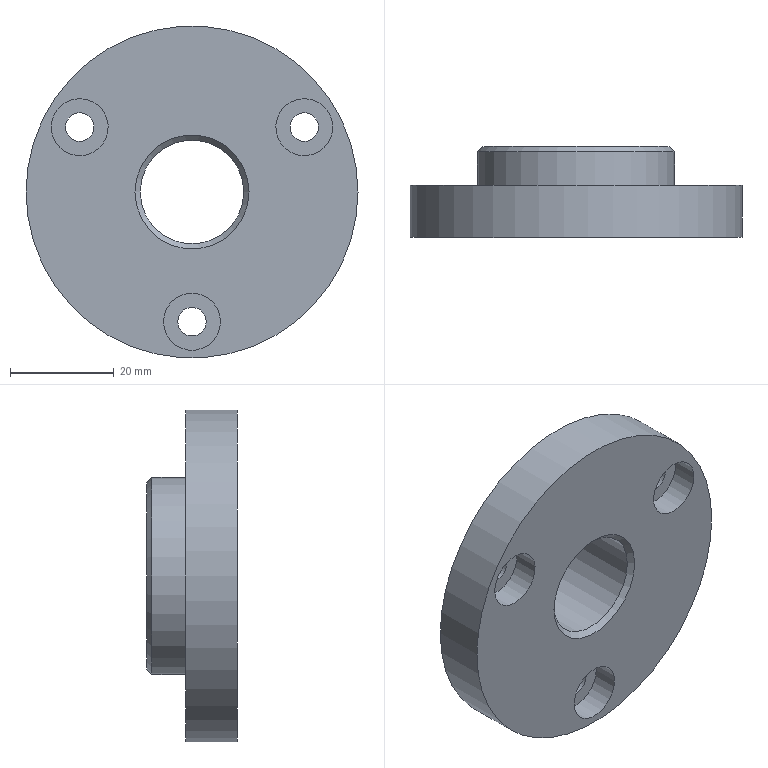Component | NX | FLANGE_COVER | 1 solid | 18 faces | box 64 x 17.5 x 64 mm | volume 33273 mm3 | cylinder 9 | plane 6 | cone 3 | commonest cylinder face diameters 11 x3 5.5 x3 64 x1 38 x1 20 x1
STEP:
#1=CARTESIAN_POINT('',(0.,0.,0.));
#2=DIRECTION('',(0.,0.,1.));
#3=DIRECTION('',(1.,0.,0.));
#4=AXIS2_PLACEMENT_3D('',#1,#2,#3);
#5=CARTESIAN_POINT('',(-127.326,-180.11,50.));
#6=VERTEX_POINT('',#5);
#7=CARTESIAN_POINT('',(-95.326,-180.11,50.));
#8=DIRECTION('',(0.,1.,0.));
#9=DIRECTION('',(-1.,0.,0.));
#10=AXIS2_PLACEMENT_3D('',#7,#8,#9);
#11=CIRCLE('',#10,32.);
#12=CARTESIAN_POINT('',(-95.326,-180.11,50.));
#13=DIRECTION('',(0.,-1.,0.));
#14=DIRECTION('',(1.,0.,0.));
#15=AXIS2_PLACEMENT_3D('',#12,#13,#14);
#16=CYLINDRICAL_SURFACE('',#15,32.);
#17=CARTESIAN_POINT('',(9.425,0.));
#18=DIRECTION('',(-1.,0.));
#19=VECTOR('',#18,1.);
#20=LINE('',#17,#19);
#21=(GEOMETRIC_REPRESENTATION_CONTEXT(2)PARAMETRIC_REPRESENTATION_CONTEXT()REPRESENTATION_CONTEXT('',''));
#22=DEFINITIONAL_REPRESENTATION('',(#20),#21);
#23=PCURVE('',#16,#22);
#24=CARTESIAN_POINT('',(-95.326,-180.11,50.));
#25=DIRECTION('',(0.,1.,0.));
#26=DIRECTION('',(-1.,0.,0.));
#27=AXIS2_PLACEMENT_3D('',#24,#25,#26);
#28=PLANE('',#27);
#29=CARTESIAN_POINT('',(0.,0.));
#30=DIRECTION('',(1.,0.));
#31=AXIS2_PLACEMENT_2D('',#29,#30);
#32=CIRCLE('',#31,32.);
#33=(GEOMETRIC_REPRESENTATION_CONTEXT(2)PARAMETRIC_REPRESENTATION_CONTEXT()REPRESENTATION_CONTEXT('',''));
#34=DEFINITIONAL_REPRESENTATION('',(#32),#33);
#35=PCURVE('',#28,#34);
#36=SURFACE_CURVE('',#11,(#23,#35),.PCURVE_S1.);
#37=EDGE_CURVE('',#6,#6,#36,.T.);
#38=ORIENTED_EDGE('',*,*,#37,.F.);
#39=CARTESIAN_POINT('',(-127.326,-190.11,50.));
#40=VERTEX_POINT('',#39);
#41=CARTESIAN_POINT('',(-127.326,-180.11,50.));
#42=CARTESIAN_POINT('',(-127.326,-190.11,50.));
#43=B_SPLINE_CURVE_WITH_KNOTS('',1,(#41,#42),.UNSPECIFIED.,.F.,.F.,(2,2),(0.,10.),.PIECEWISE_BEZIER_KNOTS.);
#44=CARTESIAN_POINT('',(9.425,0.));
#45=DIRECTION('',(0.,1.));
#46=VECTOR('',#45,1.);
#47=LINE('',#44,#46);
#48=(GEOMETRIC_REPRESENTATION_CONTEXT(2)PARAMETRIC_REPRESENTATION_CONTEXT()REPRESENTATION_CONTEXT('',''));
#49=DEFINITIONAL_REPRESENTATION('',(#47),#48);
#50=PCURVE('',#16,#49);
#51=CARTESIAN_POINT('',(3.142,0.));
#52=DIRECTION('',(0.,1.));
#53=VECTOR('',#52,1.);
#54=LINE('',#51,#53);
#55=(GEOMETRIC_REPRESENTATION_CONTEXT(2)PARAMETRIC_REPRESENTATION_CONTEXT()REPRESENTATION_CONTEXT('',''));
#56=DEFINITIONAL_REPRESENTATION('',(#54),#55);
#57=PCURVE('',#16,#56);
#58=SEAM_CURVE('',#43,(#50,#57),.PCURVE_S1.);
#59=EDGE_CURVE('',#6,#40,#58,.T.);
#60=ORIENTED_EDGE('',*,*,#59,.T.);
#61=CARTESIAN_POINT('',(-95.326,-190.11,50.));
#62=DIRECTION('',(0.,1.,0.));
#63=DIRECTION('',(-1.,0.,0.));
#64=AXIS2_PLACEMENT_3D('',#61,#62,#63);
#65=CIRCLE('',#64,32.);
#66=CARTESIAN_POINT('',(9.425,10.));
#67=DIRECTION('',(-1.,0.));
#68=VECTOR('',#67,1.);
#69=LINE('',#66,#68);
#70=(GEOMETRIC_REPRESENTATION_CONTEXT(2)PARAMETRIC_REPRESENTATION_CONTEXT()REPRESENTATION_CONTEXT('',''));
#71=DEFINITIONAL_REPRESENTATION('',(#69),#70);
#72=PCURVE('',#16,#71);
#73=CARTESIAN_POINT('',(-95.326,-190.11,50.));
#74=DIRECTION('',(0.,1.,0.));
#75=DIRECTION('',(-1.,0.,0.));
#76=AXIS2_PLACEMENT_3D('',#73,#74,#75);
#77=PLANE('',#76);
#78=CARTESIAN_POINT('',(0.,0.));
#79=DIRECTION('',(1.,0.));
#80=AXIS2_PLACEMENT_2D('',#78,#79);
#81=CIRCLE('',#80,32.);
#82=(GEOMETRIC_REPRESENTATION_CONTEXT(2)PARAMETRIC_REPRESENTATION_CONTEXT()REPRESENTATION_CONTEXT('',''));
#83=DEFINITIONAL_REPRESENTATION('',(#81),#82);
#84=PCURVE('',#77,#83);
#85=SURFACE_CURVE('',#65,(#72,#84),.PCURVE_S1.);
#86=EDGE_CURVE('',#40,#40,#85,.T.);
#87=ORIENTED_EDGE('',*,*,#86,.T.);
#88=ORIENTED_EDGE('',*,*,#59,.F.);
#89=EDGE_LOOP('',(#38,#60,#87,#88));
#90=FACE_BOUND('',#89,.T.);
#91=ADVANCED_FACE('',(#90),#16,.T.);
#92=CARTESIAN_POINT('',(-98.076,-180.11,25.));
#93=VERTEX_POINT('',#92);
#94=CARTESIAN_POINT('',(-95.326,-180.11,25.));
#95=DIRECTION('',(0.,1.,0.));
#96=DIRECTION('',(-1.,0.,0.));
#97=AXIS2_PLACEMENT_3D('',#94,#95,#96);
#98=CIRCLE('',#97,2.75);
#99=CARTESIAN_POINT('',(0.,-25.));
#100=DIRECTION('',(1.,0.));
#101=AXIS2_PLACEMENT_2D('',#99,#100);
#102=CIRCLE('',#101,2.75);
#103=(GEOMETRIC_REPRESENTATION_CONTEXT(2)PARAMETRIC_REPRESENTATION_CONTEXT()REPRESENTATION_CONTEXT('',''));
#104=DEFINITIONAL_REPRESENTATION('',(#102),#103);
#105=PCURVE('',#28,#104);
#106=CARTESIAN_POINT('',(-95.326,-148.11,25.));
#107=DIRECTION('',(0.,-1.,0.));
#108=DIRECTION('',(1.,0.,0.));
#109=AXIS2_PLACEMENT_3D('',#106,#107,#108);
#110=CYLINDRICAL_SURFACE('',#109,2.75);
#111=CARTESIAN_POINT('',(9.425,32.));
#112=DIRECTION('',(-1.,0.));
#113=VECTOR('',#112,1.);
#114=LINE('',#111,#113);
#115=(GEOMETRIC_REPRESENTATION_CONTEXT(2)PARAMETRIC_REPRESENTATION_CONTEXT()REPRESENTATION_CONTEXT('',''));
#116=DEFINITIONAL_REPRESENTATION('',(#114),#115);
#117=PCURVE('',#110,#116);
#118=SURFACE_CURVE('',#98,(#105,#117),.PCURVE_S1.);
#119=EDGE_CURVE('',#93,#93,#118,.T.);
#120=ORIENTED_EDGE('',*,*,#119,.F.);
#121=EDGE_LOOP('',(#120));
#122=FACE_BOUND('',#121,.T.);
#123=CARTESIAN_POINT('',(-76.426,-180.11,62.5));
#124=VERTEX_POINT('',#123);
#125=CARTESIAN_POINT('',(-73.676,-180.11,62.5));
#126=DIRECTION('',(0.,1.,0.));
#127=DIRECTION('',(-1.,0.,0.));
#128=AXIS2_PLACEMENT_3D('',#125,#126,#127);
#129=CIRCLE('',#128,2.75);
#130=CARTESIAN_POINT('',(-21.651,12.5));
#131=DIRECTION('',(1.,0.));
#132=AXIS2_PLACEMENT_2D('',#130,#131);
#133=CIRCLE('',#132,2.75);
#134=(GEOMETRIC_REPRESENTATION_CONTEXT(2)PARAMETRIC_REPRESENTATION_CONTEXT()REPRESENTATION_CONTEXT('',''));
#135=DEFINITIONAL_REPRESENTATION('',(#133),#134);
#136=PCURVE('',#28,#135);
#137=CARTESIAN_POINT('',(-73.676,-148.11,62.5));
#138=DIRECTION('',(0.,-1.,0.));
#139=DIRECTION('',(1.,0.,0.));
#140=AXIS2_PLACEMENT_3D('',#137,#138,#139);
#141=CYLINDRICAL_SURFACE('',#140,2.75);
#142=CARTESIAN_POINT('',(9.425,32.));
#143=DIRECTION('',(-1.,0.));
#144=VECTOR('',#143,1.);
#145=LINE('',#142,#144);
#146=(GEOMETRIC_REPRESENTATION_CONTEXT(2)PARAMETRIC_REPRESENTATION_CONTEXT()REPRESENTATION_CONTEXT('',''));
#147=DEFINITIONAL_REPRESENTATION('',(#145),#146);
#148=PCURVE('',#141,#147);
#149=SURFACE_CURVE('',#129,(#136,#148),.PCURVE_S1.);
#150=EDGE_CURVE('',#124,#124,#149,.T.);
#151=ORIENTED_EDGE('',*,*,#150,.F.);
#152=EDGE_LOOP('',(#151));
#153=FACE_BOUND('',#152,.T.);
#154=CARTESIAN_POINT('',(-119.727,-180.11,62.5));
#155=VERTEX_POINT('',#154);
#156=CARTESIAN_POINT('',(-116.977,-180.11,62.5));
#157=DIRECTION('',(0.,1.,0.));
#158=DIRECTION('',(-1.,0.,0.));
#159=AXIS2_PLACEMENT_3D('',#156,#157,#158);
#160=CIRCLE('',#159,2.75);
#161=CARTESIAN_POINT('',(21.651,12.5));
#162=DIRECTION('',(1.,0.));
#163=AXIS2_PLACEMENT_2D('',#161,#162);
#164=CIRCLE('',#163,2.75);
#165=(GEOMETRIC_REPRESENTATION_CONTEXT(2)PARAMETRIC_REPRESENTATION_CONTEXT()REPRESENTATION_CONTEXT('',''));
#166=DEFINITIONAL_REPRESENTATION('',(#164),#165);
#167=PCURVE('',#28,#166);
#168=CARTESIAN_POINT('',(-116.977,-148.11,62.5));
#169=DIRECTION('',(0.,-1.,0.));
#170=DIRECTION('',(1.,0.,0.));
#171=AXIS2_PLACEMENT_3D('',#168,#169,#170);
#172=CYLINDRICAL_SURFACE('',#171,2.75);
#173=CARTESIAN_POINT('',(9.425,32.));
#174=DIRECTION('',(-1.,0.));
#175=VECTOR('',#174,1.);
#176=LINE('',#173,#175);
#177=(GEOMETRIC_REPRESENTATION_CONTEXT(2)PARAMETRIC_REPRESENTATION_CONTEXT()REPRESENTATION_CONTEXT('',''));
#178=DEFINITIONAL_REPRESENTATION('',(#176),#177);
#179=PCURVE('',#172,#178);
#180=SURFACE_CURVE('',#160,(#167,#179),.PCURVE_S1.);
#181=EDGE_CURVE('',#155,#155,#180,.T.);
#182=ORIENTED_EDGE('',*,*,#181,.F.);
#183=EDGE_LOOP('',(#182));
#184=FACE_BOUND('',#183,.T.);
#185=CARTESIAN_POINT('',(-114.326,-180.11,50.));
#186=VERTEX_POINT('',#185);
#187=CARTESIAN_POINT('',(-95.326,-180.11,50.));
#188=DIRECTION('',(0.,1.,0.));
#189=DIRECTION('',(-1.,0.,0.));
#190=AXIS2_PLACEMENT_3D('',#187,#188,#189);
#191=CIRCLE('',#190,19.);
#192=CARTESIAN_POINT('',(0.,0.));
#193=DIRECTION('',(1.,0.));
#194=AXIS2_PLACEMENT_2D('',#192,#193);
#195=CIRCLE('',#194,19.);
#196=(GEOMETRIC_REPRESENTATION_CONTEXT(2)PARAMETRIC_REPRESENTATION_CONTEXT()REPRESENTATION_CONTEXT('',''));
#197=DEFINITIONAL_REPRESENTATION('',(#195),#196);
#198=PCURVE('',#28,#197);
#199=CARTESIAN_POINT('',(-95.326,-172.61,50.));
#200=DIRECTION('',(0.,-1.,0.));
#201=DIRECTION('',(1.,0.,0.));
#202=AXIS2_PLACEMENT_3D('',#199,#200,#201);
#203=CYLINDRICAL_SURFACE('',#202,19.);
#204=CARTESIAN_POINT('',(9.425,7.5));
#205=DIRECTION('',(-1.,0.));
#206=VECTOR('',#205,1.);
#207=LINE('',#204,#206);
#208=(GEOMETRIC_REPRESENTATION_CONTEXT(2)PARAMETRIC_REPRESENTATION_CONTEXT()REPRESENTATION_CONTEXT('',''));
#209=DEFINITIONAL_REPRESENTATION('',(#207),#208);
#210=PCURVE('',#203,#209);
#211=SURFACE_CURVE('',#191,(#198,#210),.PCURVE_S1.);
#212=EDGE_CURVE('',#186,#186,#211,.T.);
#213=ORIENTED_EDGE('',*,*,#212,.F.);
#214=EDGE_LOOP('',(#213));
#215=FACE_BOUND('',#214,.T.);
#216=ORIENTED_EDGE('',*,*,#37,.T.);
#217=EDGE_LOOP('',(#216));
#218=FACE_BOUND('',#217,.T.);
#219=ADVANCED_FACE('',(#122,#153,#184,#215,#218),#28,.T.);
#220=CARTESIAN_POINT('',(-106.326,-190.11,50.));
#221=VERTEX_POINT('',#220);
#222=CARTESIAN_POINT('',(-95.326,-190.11,50.));
#223=DIRECTION('',(0.,1.,0.));
#224=DIRECTION('',(-1.,0.,0.));
#225=AXIS2_PLACEMENT_3D('',#222,#223,#224);
#226=CIRCLE('',#225,11.);
#227=CARTESIAN_POINT('',(0.,0.));
#228=DIRECTION('',(1.,0.));
#229=AXIS2_PLACEMENT_2D('',#227,#228);
#230=CIRCLE('',#229,11.);
#231=(GEOMETRIC_REPRESENTATION_CONTEXT(2)PARAMETRIC_REPRESENTATION_CONTEXT()REPRESENTATION_CONTEXT('',''));
#232=DEFINITIONAL_REPRESENTATION('',(#230),#231);
#233=PCURVE('',#77,#232);
#234=CARTESIAN_POINT('',(-95.326,-189.11,50.));
#235=DIRECTION('',(0.,-1.,0.));
#236=DIRECTION('',(1.,0.,0.));
#237=AXIS2_PLACEMENT_3D('',#234,#235,#236);
#238=CONICAL_SURFACE('',#237,10.,0.7854);
#239=CARTESIAN_POINT('',(9.425,1.));
#240=DIRECTION('',(-1.,0.));
#241=VECTOR('',#240,1.);
#242=LINE('',#239,#241);
#243=(GEOMETRIC_REPRESENTATION_CONTEXT(2)PARAMETRIC_REPRESENTATION_CONTEXT()REPRESENTATION_CONTEXT('',''));
#244=DEFINITIONAL_REPRESENTATION('',(#242),#243);
#245=PCURVE('',#238,#244);
#246=SURFACE_CURVE('',#226,(#233,#245),.PCURVE_S1.);
#247=EDGE_CURVE('',#221,#221,#246,.T.);
#248=ORIENTED_EDGE('',*,*,#247,.T.);
#249=EDGE_LOOP('',(#248));
#250=FACE_BOUND('',#249,.T.);
#251=CARTESIAN_POINT('',(-100.826,-190.11,25.));
#252=VERTEX_POINT('',#251);
#253=CARTESIAN_POINT('',(-95.326,-190.11,25.));
#254=DIRECTION('',(0.,-1.,0.));
#255=DIRECTION('',(-1.,0.,0.));
#256=AXIS2_PLACEMENT_3D('',#253,#254,#255);
#257=CIRCLE('',#256,5.5);
#258=CARTESIAN_POINT('',(5.5,-25.));
#259=CARTESIAN_POINT('',(5.5,-34.526));
#260=CARTESIAN_POINT('',(-2.75,-29.763));
#261=CARTESIAN_POINT('',(-11.,-25.));
#262=CARTESIAN_POINT('',(-2.75,-20.237));
#263=CARTESIAN_POINT('',(5.5,-15.474));
#264=CARTESIAN_POINT('',(5.5,-25.));
#265=(BOUNDED_CURVE()B_SPLINE_CURVE(2,(#258,#259,#260,#261,#262,#263,#264),.UNSPECIFIED.,.T.,.F.)B_SPLINE_CURVE_WITH_KNOTS((1,2,2,2,2,1),(-2.094,0.,2.094,4.189,6.283,8.378),.UNSPECIFIED.)CURVE()GEOMETRIC_REPRESENTATION_ITEM()RATIONAL_B_SPLINE_CURVE((1.,0.5,1.,0.5,1.,0.5,1.))REPRESENTATION_ITEM(''));
#266=(GEOMETRIC_REPRESENTATION_CONTEXT(2)PARAMETRIC_REPRESENTATION_CONTEXT()REPRESENTATION_CONTEXT('',''));
#267=DEFINITIONAL_REPRESENTATION('',(#265),#266);
#268=PCURVE('',#77,#267);
#269=CARTESIAN_POINT('',(-95.326,-185.11,25.));
#270=DIRECTION('',(0.,-1.,0.));
#271=DIRECTION('',(1.,0.,0.));
#272=AXIS2_PLACEMENT_3D('',#269,#270,#271);
#273=CYLINDRICAL_SURFACE('',#272,5.5);
#274=CARTESIAN_POINT('',(3.142,5.));
#275=DIRECTION('',(1.,0.));
#276=VECTOR('',#275,1.);
#277=LINE('',#274,#276);
#278=(GEOMETRIC_REPRESENTATION_CONTEXT(2)PARAMETRIC_REPRESENTATION_CONTEXT()REPRESENTATION_CONTEXT('',''));
#279=DEFINITIONAL_REPRESENTATION('',(#277),#278);
#280=PCURVE('',#273,#279);
#281=SURFACE_CURVE('',#257,(#268,#280),.PCURVE_S1.);
#282=EDGE_CURVE('',#252,#252,#281,.T.);
#283=ORIENTED_EDGE('',*,*,#282,.F.);
#284=EDGE_LOOP('',(#283));
#285=FACE_BOUND('',#284,.T.);
#286=CARTESIAN_POINT('',(-70.926,-190.11,57.737));
#287=VERTEX_POINT('',#286);
#288=CARTESIAN_POINT('',(-73.676,-190.11,62.5));
#289=DIRECTION('',(0.,-1.,0.));
#290=DIRECTION('',(0.5,0.,-0.866));
#291=AXIS2_PLACEMENT_3D('',#288,#289,#290);
#292=CIRCLE('',#291,5.5);
#293=CARTESIAN_POINT('',(-24.401,7.737));
#294=CARTESIAN_POINT('',(-32.651,12.5));
#295=CARTESIAN_POINT('',(-24.401,17.263));
#296=CARTESIAN_POINT('',(-16.151,22.026));
#297=CARTESIAN_POINT('',(-16.151,12.5));
#298=CARTESIAN_POINT('',(-16.151,2.974));
#299=CARTESIAN_POINT('',(-24.401,7.737));
#300=(BOUNDED_CURVE()B_SPLINE_CURVE(2,(#293,#294,#295,#296,#297,#298,#299),.UNSPECIFIED.,.T.,.F.)B_SPLINE_CURVE_WITH_KNOTS((1,2,2,2,2,1),(-2.094,0.,2.094,4.189,6.283,8.378),.UNSPECIFIED.)CURVE()GEOMETRIC_REPRESENTATION_ITEM()RATIONAL_B_SPLINE_CURVE((1.,0.5,1.,0.5,1.,0.5,1.))REPRESENTATION_ITEM(''));
#301=(GEOMETRIC_REPRESENTATION_CONTEXT(2)PARAMETRIC_REPRESENTATION_CONTEXT()REPRESENTATION_CONTEXT('',''));
#302=DEFINITIONAL_REPRESENTATION('',(#300),#301);
#303=PCURVE('',#77,#302);
#304=CARTESIAN_POINT('',(-73.676,-185.11,62.5));
#305=DIRECTION('',(0.,-1.,0.));
#306=DIRECTION('',(1.,0.,0.));
#307=AXIS2_PLACEMENT_3D('',#304,#305,#306);
#308=CYLINDRICAL_SURFACE('',#307,5.5);
#309=CARTESIAN_POINT('',(5.236,5.));
#310=DIRECTION('',(1.,0.));
#311=VECTOR('',#310,1.);
#312=LINE('',#309,#311);
#313=(GEOMETRIC_REPRESENTATION_CONTEXT(2)PARAMETRIC_REPRESENTATION_CONTEXT()REPRESENTATION_CONTEXT('',''));
#314=DEFINITIONAL_REPRESENTATION('',(#312),#313);
#315=PCURVE('',#308,#314);
#316=SURFACE_CURVE('',#292,(#303,#315),.PCURVE_S1.);
#317=EDGE_CURVE('',#287,#287,#316,.T.);
#318=ORIENTED_EDGE('',*,*,#317,.F.);
#319=EDGE_LOOP('',(#318));
#320=FACE_BOUND('',#319,.T.);
#321=CARTESIAN_POINT('',(-114.227,-190.11,67.263));
#322=VERTEX_POINT('',#321);
#323=CARTESIAN_POINT('',(-116.977,-190.11,62.5));
#324=DIRECTION('',(0.,-1.,0.));
#325=DIRECTION('',(0.5,0.,0.866));
#326=AXIS2_PLACEMENT_3D('',#323,#324,#325);
#327=CIRCLE('',#326,5.5);
#328=CARTESIAN_POINT('',(18.901,17.263));
#329=CARTESIAN_POINT('',(27.151,22.026));
#330=CARTESIAN_POINT('',(27.151,12.5));
#331=CARTESIAN_POINT('',(27.151,2.974));
#332=CARTESIAN_POINT('',(18.901,7.737));
#333=CARTESIAN_POINT('',(10.651,12.5));
#334=CARTESIAN_POINT('',(18.901,17.263));
#335=(BOUNDED_CURVE()B_SPLINE_CURVE(2,(#328,#329,#330,#331,#332,#333,#334),.UNSPECIFIED.,.T.,.F.)B_SPLINE_CURVE_WITH_KNOTS((1,2,2,2,2,1),(-2.094,0.,2.094,4.189,6.283,8.378),.UNSPECIFIED.)CURVE()GEOMETRIC_REPRESENTATION_ITEM()RATIONAL_B_SPLINE_CURVE((1.,0.5,1.,0.5,1.,0.5,1.))REPRESENTATION_ITEM(''));
#336=(GEOMETRIC_REPRESENTATION_CONTEXT(2)PARAMETRIC_REPRESENTATION_CONTEXT()REPRESENTATION_CONTEXT('',''));
#337=DEFINITIONAL_REPRESENTATION('',(#335),#336);
#338=PCURVE('',#77,#337);
#339=CARTESIAN_POINT('',(-116.977,-185.11,62.5));
#340=DIRECTION('',(0.,-1.,0.));
#341=DIRECTION('',(1.,0.,0.));
#342=AXIS2_PLACEMENT_3D('',#339,#340,#341);
#343=CYLINDRICAL_SURFACE('',#342,5.5);
#344=CARTESIAN_POINT('',(1.047,5.));
#345=DIRECTION('',(1.,0.));
#346=VECTOR('',#345,1.);
#347=LINE('',#344,#346);
#348=(GEOMETRIC_REPRESENTATION_CONTEXT(2)PARAMETRIC_REPRESENTATION_CONTEXT()REPRESENTATION_CONTEXT('',''));
#349=DEFINITIONAL_REPRESENTATION('',(#347),#348);
#350=PCURVE('',#343,#349);
#351=SURFACE_CURVE('',#327,(#338,#350),.PCURVE_S1.);
#352=EDGE_CURVE('',#322,#322,#351,.T.);
#353=ORIENTED_EDGE('',*,*,#352,.F.);
#354=EDGE_LOOP('',(#353));
#355=FACE_BOUND('',#354,.T.);
#356=ORIENTED_EDGE('',*,*,#86,.F.);
#357=EDGE_LOOP('',(#356));
#358=FACE_BOUND('',#357,.T.);
#359=ADVANCED_FACE('',(#250,#285,#320,#355,#358),#77,.F.);
#360=CARTESIAN_POINT('',(-114.326,-173.61,50.));
#361=VERTEX_POINT('',#360);
#362=CARTESIAN_POINT('',(-95.326,-173.61,50.));
#363=DIRECTION('',(0.,-1.,0.));
#364=DIRECTION('',(-1.,0.,0.));
#365=AXIS2_PLACEMENT_3D('',#362,#363,#364);
#366=CIRCLE('',#365,19.);
#367=CARTESIAN_POINT('',(3.142,1.));
#368=DIRECTION('',(1.,0.));
#369=VECTOR('',#368,1.);
#370=LINE('',#367,#369);
#371=(GEOMETRIC_REPRESENTATION_CONTEXT(2)PARAMETRIC_REPRESENTATION_CONTEXT()REPRESENTATION_CONTEXT('',''));
#372=DEFINITIONAL_REPRESENTATION('',(#370),#371);
#373=PCURVE('',#203,#372);
#374=CARTESIAN_POINT('',(-95.326,-172.61,50.));
#375=DIRECTION('',(0.,-1.,0.));
#376=DIRECTION('',(1.,0.,0.));
#377=AXIS2_PLACEMENT_3D('',#374,#375,#376);
#378=CONICAL_SURFACE('',#377,18.,0.7854);
#379=CARTESIAN_POINT('',(3.142,1.));
#380=DIRECTION('',(1.,0.));
#381=VECTOR('',#380,1.);
#382=LINE('',#379,#381);
#383=(GEOMETRIC_REPRESENTATION_CONTEXT(2)PARAMETRIC_REPRESENTATION_CONTEXT()REPRESENTATION_CONTEXT('',''));
#384=DEFINITIONAL_REPRESENTATION('',(#382),#383);
#385=PCURVE('',#378,#384);
#386=SURFACE_CURVE('',#366,(#373,#385),.PCURVE_S1.);
#387=EDGE_CURVE('',#361,#361,#386,.T.);
#388=ORIENTED_EDGE('',*,*,#387,.T.);
#389=CARTESIAN_POINT('',(-114.326,-173.61,50.));
#390=CARTESIAN_POINT('',(-114.326,-180.11,50.));
#391=B_SPLINE_CURVE_WITH_KNOTS('',1,(#389,#390),.UNSPECIFIED.,.F.,.F.,(2,2),(1.,7.5),.PIECEWISE_BEZIER_KNOTS.);
#392=CARTESIAN_POINT('',(9.425,0.));
#393=DIRECTION('',(0.,1.));
#394=VECTOR('',#393,1.);
#395=LINE('',#392,#394);
#396=(GEOMETRIC_REPRESENTATION_CONTEXT(2)PARAMETRIC_REPRESENTATION_CONTEXT()REPRESENTATION_CONTEXT('',''));
#397=DEFINITIONAL_REPRESENTATION('',(#395),#396);
#398=PCURVE('',#203,#397);
#399=CARTESIAN_POINT('',(3.142,0.));
#400=DIRECTION('',(0.,1.));
#401=VECTOR('',#400,1.);
#402=LINE('',#399,#401);
#403=(GEOMETRIC_REPRESENTATION_CONTEXT(2)PARAMETRIC_REPRESENTATION_CONTEXT()REPRESENTATION_CONTEXT('',''));
#404=DEFINITIONAL_REPRESENTATION('',(#402),#403);
#405=PCURVE('',#203,#404);
#406=SEAM_CURVE('',#391,(#398,#405),.PCURVE_S1.);
#407=EDGE_CURVE('',#361,#186,#406,.T.);
#408=ORIENTED_EDGE('',*,*,#407,.T.);
#409=ORIENTED_EDGE('',*,*,#212,.T.);
#410=ORIENTED_EDGE('',*,*,#407,.F.);
#411=EDGE_LOOP('',(#388,#408,#409,#410));
#412=FACE_BOUND('',#411,.T.);
#413=ADVANCED_FACE('',(#412),#203,.T.);
#414=CARTESIAN_POINT('',(-113.326,-172.61,50.));
#415=VERTEX_POINT('',#414);
#416=CARTESIAN_POINT('',(-95.326,-172.61,50.));
#417=DIRECTION('',(0.,1.,0.));
#418=DIRECTION('',(-1.,0.,0.));
#419=AXIS2_PLACEMENT_3D('',#416,#417,#418);
#420=CIRCLE('',#419,18.);
#421=CARTESIAN_POINT('',(-95.326,-172.61,50.));
#422=DIRECTION('',(0.,1.,0.));
#423=DIRECTION('',(-1.,0.,0.));
#424=AXIS2_PLACEMENT_3D('',#421,#422,#423);
#425=PLANE('',#424);
#426=CARTESIAN_POINT('',(0.,0.));
#427=DIRECTION('',(1.,0.));
#428=AXIS2_PLACEMENT_2D('',#426,#427);
#429=CIRCLE('',#428,18.);
#430=(GEOMETRIC_REPRESENTATION_CONTEXT(2)PARAMETRIC_REPRESENTATION_CONTEXT()REPRESENTATION_CONTEXT('',''));
#431=DEFINITIONAL_REPRESENTATION('',(#429),#430);
#432=PCURVE('',#425,#431);
#433=CARTESIAN_POINT('',(9.425,0.));
#434=DIRECTION('',(-1.,0.));
#435=VECTOR('',#434,1.);
#436=LINE('',#433,#435);
#437=(GEOMETRIC_REPRESENTATION_CONTEXT(2)PARAMETRIC_REPRESENTATION_CONTEXT()REPRESENTATION_CONTEXT('',''));
#438=DEFINITIONAL_REPRESENTATION('',(#436),#437);
#439=PCURVE('',#378,#438);
#440=SURFACE_CURVE('',#420,(#432,#439),.PCURVE_S1.);
#441=EDGE_CURVE('',#415,#415,#440,.T.);
#442=ORIENTED_EDGE('',*,*,#441,.T.);
#443=EDGE_LOOP('',(#442));
#444=FACE_BOUND('',#443,.T.);
#445=CARTESIAN_POINT('',(-106.326,-172.61,50.));
#446=VERTEX_POINT('',#445);
#447=CARTESIAN_POINT('',(-95.326,-172.61,50.));
#448=DIRECTION('',(0.,-1.,0.));
#449=DIRECTION('',(-1.,0.,0.));
#450=AXIS2_PLACEMENT_3D('',#447,#448,#449);
#451=CIRCLE('',#450,11.);
#452=CARTESIAN_POINT('',(11.,0.));
#453=CARTESIAN_POINT('',(11.,-19.053));
#454=CARTESIAN_POINT('',(-5.5,-9.526));
#455=CARTESIAN_POINT('',(-22.,-0.));
#456=CARTESIAN_POINT('',(-5.5,9.526));
#457=CARTESIAN_POINT('',(11.,19.053));
#458=CARTESIAN_POINT('',(11.,0.));
#459=(BOUNDED_CURVE()B_SPLINE_CURVE(2,(#452,#453,#454,#455,#456,#457,#458),.UNSPECIFIED.,.T.,.F.)B_SPLINE_CURVE_WITH_KNOTS((1,2,2,2,2,1),(-2.094,0.,2.094,4.189,6.283,8.378),.UNSPECIFIED.)CURVE()GEOMETRIC_REPRESENTATION_ITEM()RATIONAL_B_SPLINE_CURVE((1.,0.5,1.,0.5,1.,0.5,1.))REPRESENTATION_ITEM(''));
#460=(GEOMETRIC_REPRESENTATION_CONTEXT(2)PARAMETRIC_REPRESENTATION_CONTEXT()REPRESENTATION_CONTEXT('',''));
#461=DEFINITIONAL_REPRESENTATION('',(#459),#460);
#462=PCURVE('',#425,#461);
#463=CARTESIAN_POINT('',(-95.326,-173.61,50.));
#464=DIRECTION('',(0.,1.,0.));
#465=DIRECTION('',(-1.,0.,0.));
#466=AXIS2_PLACEMENT_3D('',#463,#464,#465);
#467=CONICAL_SURFACE('',#466,10.,0.7854);
#468=CARTESIAN_POINT('',(6.283,1.));
#469=DIRECTION('',(-1.,0.));
#470=VECTOR('',#469,1.);
#471=LINE('',#468,#470);
#472=(GEOMETRIC_REPRESENTATION_CONTEXT(2)PARAMETRIC_REPRESENTATION_CONTEXT()REPRESENTATION_CONTEXT('',''));
#473=DEFINITIONAL_REPRESENTATION('',(#471),#472);
#474=PCURVE('',#467,#473);
#475=SURFACE_CURVE('',#451,(#462,#474),.PCURVE_S1.);
#476=EDGE_CURVE('',#446,#446,#475,.T.);
#477=ORIENTED_EDGE('',*,*,#476,.T.);
#478=EDGE_LOOP('',(#477));
#479=FACE_BOUND('',#478,.T.);
#480=ADVANCED_FACE('',(#444,#479),#425,.T.);
#481=CARTESIAN_POINT('',(-114.227,-185.11,67.263));
#482=VERTEX_POINT('',#481);
#483=CARTESIAN_POINT('',(-116.977,-185.11,62.5));
#484=DIRECTION('',(0.,1.,0.));
#485=DIRECTION('',(0.5,0.,0.866));
#486=AXIS2_PLACEMENT_3D('',#483,#484,#485);
#487=CIRCLE('',#486,5.5);
#488=CARTESIAN_POINT('',(7.33,0.));
#489=DIRECTION('',(-1.,0.));
#490=VECTOR('',#489,1.);
#491=LINE('',#488,#490);
#492=(GEOMETRIC_REPRESENTATION_CONTEXT(2)PARAMETRIC_REPRESENTATION_CONTEXT()REPRESENTATION_CONTEXT('',''));
#493=DEFINITIONAL_REPRESENTATION('',(#491),#492);
#494=PCURVE('',#343,#493);
#495=CARTESIAN_POINT('',(-116.977,-185.11,62.5));
#496=DIRECTION('',(0.,-1.,0.));
#497=DIRECTION('',(1.,0.,0.));
#498=AXIS2_PLACEMENT_3D('',#495,#496,#497);
#499=PLANE('',#498);
#500=CARTESIAN_POINT('',(2.75,4.763));
#501=CARTESIAN_POINT('',(11.,-0.));
#502=CARTESIAN_POINT('',(2.75,-4.763));
#503=CARTESIAN_POINT('',(-5.5,-9.526));
#504=CARTESIAN_POINT('',(-5.5,0.));
#505=CARTESIAN_POINT('',(-5.5,9.526));
#506=CARTESIAN_POINT('',(2.75,4.763));
#507=(BOUNDED_CURVE()B_SPLINE_CURVE(2,(#500,#501,#502,#503,#504,#505,#506),.UNSPECIFIED.,.T.,.F.)B_SPLINE_CURVE_WITH_KNOTS((1,2,2,2,2,1),(-2.094,0.,2.094,4.189,6.283,8.378),.UNSPECIFIED.)CURVE()GEOMETRIC_REPRESENTATION_ITEM()RATIONAL_B_SPLINE_CURVE((1.,0.5,1.,0.5,1.,0.5,1.))REPRESENTATION_ITEM(''));
#508=(GEOMETRIC_REPRESENTATION_CONTEXT(2)PARAMETRIC_REPRESENTATION_CONTEXT()REPRESENTATION_CONTEXT('',''));
#509=DEFINITIONAL_REPRESENTATION('',(#507),#508);
#510=PCURVE('',#499,#509);
#511=SURFACE_CURVE('',#487,(#494,#510),.PCURVE_S1.);
#512=EDGE_CURVE('',#482,#482,#511,.T.);
#513=ORIENTED_EDGE('',*,*,#512,.F.);
#514=CARTESIAN_POINT('',(-114.227,-185.11,67.263));
#515=CARTESIAN_POINT('',(-114.227,-190.11,67.263));
#516=B_SPLINE_CURVE_WITH_KNOTS('',1,(#514,#515),.UNSPECIFIED.,.F.,.F.,(2,2),(0.,5.),.PIECEWISE_BEZIER_KNOTS.);
#517=CARTESIAN_POINT('',(7.33,0.));
#518=DIRECTION('',(0.,1.));
#519=VECTOR('',#518,1.);
#520=LINE('',#517,#519);
#521=(GEOMETRIC_REPRESENTATION_CONTEXT(2)PARAMETRIC_REPRESENTATION_CONTEXT()REPRESENTATION_CONTEXT('',''));
#522=DEFINITIONAL_REPRESENTATION('',(#520),#521);
#523=PCURVE('',#343,#522);
#524=CARTESIAN_POINT('',(1.047,0.));
#525=DIRECTION('',(0.,1.));
#526=VECTOR('',#525,1.);
#527=LINE('',#524,#526);
#528=(GEOMETRIC_REPRESENTATION_CONTEXT(2)PARAMETRIC_REPRESENTATION_CONTEXT()REPRESENTATION_CONTEXT('',''));
#529=DEFINITIONAL_REPRESENTATION('',(#527),#528);
#530=PCURVE('',#343,#529);
#531=SEAM_CURVE('',#516,(#523,#530),.PCURVE_S1.);
#532=EDGE_CURVE('',#482,#322,#531,.T.);
#533=ORIENTED_EDGE('',*,*,#532,.T.);
#534=ORIENTED_EDGE('',*,*,#352,.F.);
#535=ORIENTED_EDGE('',*,*,#532,.F.);
#536=EDGE_LOOP('',(#513,#533,#534,#535));
#537=FACE_BOUND('',#536,.F.);
#538=ADVANCED_FACE('',(#537),#343,.F.);
#539=CARTESIAN_POINT('',(-119.727,-185.11,62.5));
#540=VERTEX_POINT('',#539);
#541=CARTESIAN_POINT('',(-116.977,-185.11,62.5));
#542=DIRECTION('',(0.,-1.,0.));
#543=DIRECTION('',(-1.,0.,0.));
#544=AXIS2_PLACEMENT_3D('',#541,#542,#543);
#545=CIRCLE('',#544,2.75);
#546=CARTESIAN_POINT('',(0.,0.));
#547=DIRECTION('',(-1.,0.));
#548=AXIS2_PLACEMENT_2D('',#546,#547);
#549=CIRCLE('',#548,2.75);
#550=(GEOMETRIC_REPRESENTATION_CONTEXT(2)PARAMETRIC_REPRESENTATION_CONTEXT()REPRESENTATION_CONTEXT('',''));
#551=DEFINITIONAL_REPRESENTATION('',(#549),#550);
#552=PCURVE('',#499,#551);
#553=CARTESIAN_POINT('',(3.142,37.));
#554=DIRECTION('',(1.,0.));
#555=VECTOR('',#554,1.);
#556=LINE('',#553,#555);
#557=(GEOMETRIC_REPRESENTATION_CONTEXT(2)PARAMETRIC_REPRESENTATION_CONTEXT()REPRESENTATION_CONTEXT('',''));
#558=DEFINITIONAL_REPRESENTATION('',(#556),#557);
#559=PCURVE('',#172,#558);
#560=SURFACE_CURVE('',#545,(#552,#559),.PCURVE_S1.);
#561=EDGE_CURVE('',#540,#540,#560,.T.);
#562=ORIENTED_EDGE('',*,*,#561,.F.);
#563=EDGE_LOOP('',(#562));
#564=FACE_BOUND('',#563,.T.);
#565=ORIENTED_EDGE('',*,*,#512,.F.);
#566=EDGE_LOOP('',(#565));
#567=FACE_BOUND('',#566,.T.);
#568=ADVANCED_FACE('',(#564,#567),#499,.T.);
#569=CARTESIAN_POINT('',(-70.926,-185.11,57.737));
#570=VERTEX_POINT('',#569);
#571=CARTESIAN_POINT('',(-73.676,-185.11,62.5));
#572=DIRECTION('',(0.,1.,0.));
#573=DIRECTION('',(0.5,0.,-0.866));
#574=AXIS2_PLACEMENT_3D('',#571,#572,#573);
#575=CIRCLE('',#574,5.5);
#576=CARTESIAN_POINT('',(11.519,0.));
#577=DIRECTION('',(-1.,0.));
#578=VECTOR('',#577,1.);
#579=LINE('',#576,#578);
#580=(GEOMETRIC_REPRESENTATION_CONTEXT(2)PARAMETRIC_REPRESENTATION_CONTEXT()REPRESENTATION_CONTEXT('',''));
#581=DEFINITIONAL_REPRESENTATION('',(#579),#580);
#582=PCURVE('',#308,#581);
#583=CARTESIAN_POINT('',(-73.676,-185.11,62.5));
#584=DIRECTION('',(0.,-1.,0.));
#585=DIRECTION('',(1.,0.,0.));
#586=AXIS2_PLACEMENT_3D('',#583,#584,#585);
#587=PLANE('',#586);
#588=CARTESIAN_POINT('',(2.75,-4.763));
#589=CARTESIAN_POINT('',(-5.5,-9.526));
#590=CARTESIAN_POINT('',(-5.5,0.));
#591=CARTESIAN_POINT('',(-5.5,9.526));
#592=CARTESIAN_POINT('',(2.75,4.763));
#593=CARTESIAN_POINT('',(11.,-0.));
#594=CARTESIAN_POINT('',(2.75,-4.763));
#595=(BOUNDED_CURVE()B_SPLINE_CURVE(2,(#588,#589,#590,#591,#592,#593,#594),.UNSPECIFIED.,.T.,.F.)B_SPLINE_CURVE_WITH_KNOTS((1,2,2,2,2,1),(-2.094,0.,2.094,4.189,6.283,8.378),.UNSPECIFIED.)CURVE()GEOMETRIC_REPRESENTATION_ITEM()RATIONAL_B_SPLINE_CURVE((1.,0.5,1.,0.5,1.,0.5,1.))REPRESENTATION_ITEM(''));
#596=(GEOMETRIC_REPRESENTATION_CONTEXT(2)PARAMETRIC_REPRESENTATION_CONTEXT()REPRESENTATION_CONTEXT('',''));
#597=DEFINITIONAL_REPRESENTATION('',(#595),#596);
#598=PCURVE('',#587,#597);
#599=SURFACE_CURVE('',#575,(#582,#598),.PCURVE_S1.);
#600=EDGE_CURVE('',#570,#570,#599,.T.);
#601=ORIENTED_EDGE('',*,*,#600,.F.);
#602=CARTESIAN_POINT('',(-70.926,-185.11,57.737));
#603=CARTESIAN_POINT('',(-70.926,-190.11,57.737));
#604=B_SPLINE_CURVE_WITH_KNOTS('',1,(#602,#603),.UNSPECIFIED.,.F.,.F.,(2,2),(0.,5.),.PIECEWISE_BEZIER_KNOTS.);
#605=CARTESIAN_POINT('',(11.519,0.));
#606=DIRECTION('',(0.,1.));
#607=VECTOR('',#606,1.);
#608=LINE('',#605,#607);
#609=(GEOMETRIC_REPRESENTATION_CONTEXT(2)PARAMETRIC_REPRESENTATION_CONTEXT()REPRESENTATION_CONTEXT('',''));
#610=DEFINITIONAL_REPRESENTATION('',(#608),#609);
#611=PCURVE('',#308,#610);
#612=CARTESIAN_POINT('',(5.236,0.));
#613=DIRECTION('',(0.,1.));
#614=VECTOR('',#613,1.);
#615=LINE('',#612,#614);
#616=(GEOMETRIC_REPRESENTATION_CONTEXT(2)PARAMETRIC_REPRESENTATION_CONTEXT()REPRESENTATION_CONTEXT('',''));
#617=DEFINITIONAL_REPRESENTATION('',(#615),#616);
#618=PCURVE('',#308,#617);
#619=SEAM_CURVE('',#604,(#611,#618),.PCURVE_S1.);
#620=EDGE_CURVE('',#570,#287,#619,.T.);
#621=ORIENTED_EDGE('',*,*,#620,.T.);
#622=ORIENTED_EDGE('',*,*,#317,.F.);
#623=ORIENTED_EDGE('',*,*,#620,.F.);
#624=EDGE_LOOP('',(#601,#621,#622,#623));
#625=FACE_BOUND('',#624,.F.);
#626=ADVANCED_FACE('',(#625),#308,.F.);
#627=CARTESIAN_POINT('',(-76.426,-185.11,62.5));
#628=VERTEX_POINT('',#627);
#629=CARTESIAN_POINT('',(-73.676,-185.11,62.5));
#630=DIRECTION('',(0.,-1.,0.));
#631=DIRECTION('',(-1.,0.,0.));
#632=AXIS2_PLACEMENT_3D('',#629,#630,#631);
#633=CIRCLE('',#632,2.75);
#634=CARTESIAN_POINT('',(0.,0.));
#635=DIRECTION('',(-1.,0.));
#636=AXIS2_PLACEMENT_2D('',#634,#635);
#637=CIRCLE('',#636,2.75);
#638=(GEOMETRIC_REPRESENTATION_CONTEXT(2)PARAMETRIC_REPRESENTATION_CONTEXT()REPRESENTATION_CONTEXT('',''));
#639=DEFINITIONAL_REPRESENTATION('',(#637),#638);
#640=PCURVE('',#587,#639);
#641=CARTESIAN_POINT('',(3.142,37.));
#642=DIRECTION('',(1.,0.));
#643=VECTOR('',#642,1.);
#644=LINE('',#641,#643);
#645=(GEOMETRIC_REPRESENTATION_CONTEXT(2)PARAMETRIC_REPRESENTATION_CONTEXT()REPRESENTATION_CONTEXT('',''));
#646=DEFINITIONAL_REPRESENTATION('',(#644),#645);
#647=PCURVE('',#141,#646);
#648=SURFACE_CURVE('',#633,(#640,#647),.PCURVE_S1.);
#649=EDGE_CURVE('',#628,#628,#648,.T.);
#650=ORIENTED_EDGE('',*,*,#649,.F.);
#651=EDGE_LOOP('',(#650));
#652=FACE_BOUND('',#651,.T.);
#653=ORIENTED_EDGE('',*,*,#600,.F.);
#654=EDGE_LOOP('',(#653));
#655=FACE_BOUND('',#654,.T.);
#656=ADVANCED_FACE('',(#652,#655),#587,.T.);
#657=CARTESIAN_POINT('',(-100.826,-185.11,25.));
#658=VERTEX_POINT('',#657);
#659=CARTESIAN_POINT('',(-95.326,-185.11,25.));
#660=DIRECTION('',(0.,1.,0.));
#661=DIRECTION('',(-1.,0.,0.));
#662=AXIS2_PLACEMENT_3D('',#659,#660,#661);
#663=CIRCLE('',#662,5.5);
#664=CARTESIAN_POINT('',(9.425,0.));
#665=DIRECTION('',(-1.,0.));
#666=VECTOR('',#665,1.);
#667=LINE('',#664,#666);
#668=(GEOMETRIC_REPRESENTATION_CONTEXT(2)PARAMETRIC_REPRESENTATION_CONTEXT()REPRESENTATION_CONTEXT('',''));
#669=DEFINITIONAL_REPRESENTATION('',(#667),#668);
#670=PCURVE('',#273,#669);
#671=CARTESIAN_POINT('',(-95.326,-185.11,25.));
#672=DIRECTION('',(0.,-1.,0.));
#673=DIRECTION('',(1.,0.,0.));
#674=AXIS2_PLACEMENT_3D('',#671,#672,#673);
#675=PLANE('',#674);
#676=CARTESIAN_POINT('',(-5.5,0.));
#677=CARTESIAN_POINT('',(-5.5,9.526));
#678=CARTESIAN_POINT('',(2.75,4.763));
#679=CARTESIAN_POINT('',(11.,0.));
#680=CARTESIAN_POINT('',(2.75,-4.763));
#681=CARTESIAN_POINT('',(-5.5,-9.526));
#682=CARTESIAN_POINT('',(-5.5,0.));
#683=(BOUNDED_CURVE()B_SPLINE_CURVE(2,(#676,#677,#678,#679,#680,#681,#682),.UNSPECIFIED.,.T.,.F.)B_SPLINE_CURVE_WITH_KNOTS((1,2,2,2,2,1),(-2.094,0.,2.094,4.189,6.283,8.378),.UNSPECIFIED.)CURVE()GEOMETRIC_REPRESENTATION_ITEM()RATIONAL_B_SPLINE_CURVE((1.,0.5,1.,0.5,1.,0.5,1.))REPRESENTATION_ITEM(''));
#684=(GEOMETRIC_REPRESENTATION_CONTEXT(2)PARAMETRIC_REPRESENTATION_CONTEXT()REPRESENTATION_CONTEXT('',''));
#685=DEFINITIONAL_REPRESENTATION('',(#683),#684);
#686=PCURVE('',#675,#685);
#687=SURFACE_CURVE('',#663,(#670,#686),.PCURVE_S1.);
#688=EDGE_CURVE('',#658,#658,#687,.T.);
#689=ORIENTED_EDGE('',*,*,#688,.F.);
#690=CARTESIAN_POINT('',(-100.826,-185.11,25.));
#691=CARTESIAN_POINT('',(-100.826,-190.11,25.));
#692=B_SPLINE_CURVE_WITH_KNOTS('',1,(#690,#691),.UNSPECIFIED.,.F.,.F.,(2,2),(0.,5.),.PIECEWISE_BEZIER_KNOTS.);
#693=CARTESIAN_POINT('',(9.425,0.));
#694=DIRECTION('',(0.,1.));
#695=VECTOR('',#694,1.);
#696=LINE('',#693,#695);
#697=(GEOMETRIC_REPRESENTATION_CONTEXT(2)PARAMETRIC_REPRESENTATION_CONTEXT()REPRESENTATION_CONTEXT('',''));
#698=DEFINITIONAL_REPRESENTATION('',(#696),#697);
#699=PCURVE('',#273,#698);
#700=CARTESIAN_POINT('',(3.142,0.));
#701=DIRECTION('',(0.,1.));
#702=VECTOR('',#701,1.);
#703=LINE('',#700,#702);
#704=(GEOMETRIC_REPRESENTATION_CONTEXT(2)PARAMETRIC_REPRESENTATION_CONTEXT()REPRESENTATION_CONTEXT('',''));
#705=DEFINITIONAL_REPRESENTATION('',(#703),#704);
#706=PCURVE('',#273,#705);
#707=SEAM_CURVE('',#692,(#699,#706),.PCURVE_S1.);
#708=EDGE_CURVE('',#658,#252,#707,.T.);
#709=ORIENTED_EDGE('',*,*,#708,.T.);
#710=ORIENTED_EDGE('',*,*,#282,.F.);
#711=ORIENTED_EDGE('',*,*,#708,.F.);
#712=EDGE_LOOP('',(#689,#709,#710,#711));
#713=FACE_BOUND('',#712,.F.);
#714=ADVANCED_FACE('',(#713),#273,.F.);
#715=CARTESIAN_POINT('',(-98.076,-185.11,25.));
#716=VERTEX_POINT('',#715);
#717=CARTESIAN_POINT('',(-95.326,-185.11,25.));
#718=DIRECTION('',(0.,-1.,0.));
#719=DIRECTION('',(-1.,0.,0.));
#720=AXIS2_PLACEMENT_3D('',#717,#718,#719);
#721=CIRCLE('',#720,2.75);
#722=CARTESIAN_POINT('',(0.,0.));
#723=DIRECTION('',(-1.,0.));
#724=AXIS2_PLACEMENT_2D('',#722,#723);
#725=CIRCLE('',#724,2.75);
#726=(GEOMETRIC_REPRESENTATION_CONTEXT(2)PARAMETRIC_REPRESENTATION_CONTEXT()REPRESENTATION_CONTEXT('',''));
#727=DEFINITIONAL_REPRESENTATION('',(#725),#726);
#728=PCURVE('',#675,#727);
#729=CARTESIAN_POINT('',(3.142,37.));
#730=DIRECTION('',(1.,0.));
#731=VECTOR('',#730,1.);
#732=LINE('',#729,#731);
#733=(GEOMETRIC_REPRESENTATION_CONTEXT(2)PARAMETRIC_REPRESENTATION_CONTEXT()REPRESENTATION_CONTEXT('',''));
#734=DEFINITIONAL_REPRESENTATION('',(#732),#733);
#735=PCURVE('',#110,#734);
#736=SURFACE_CURVE('',#721,(#728,#735),.PCURVE_S1.);
#737=EDGE_CURVE('',#716,#716,#736,.T.);
#738=ORIENTED_EDGE('',*,*,#737,.F.);
#739=EDGE_LOOP('',(#738));
#740=FACE_BOUND('',#739,.T.);
#741=ORIENTED_EDGE('',*,*,#688,.F.);
#742=EDGE_LOOP('',(#741));
#743=FACE_BOUND('',#742,.T.);
#744=ADVANCED_FACE('',(#740,#743),#675,.T.);
#745=ORIENTED_EDGE('',*,*,#181,.F.);
#746=CARTESIAN_POINT('',(-119.727,-180.11,62.5));
#747=CARTESIAN_POINT('',(-119.727,-185.11,62.5));
#748=B_SPLINE_CURVE_WITH_KNOTS('',1,(#746,#747),.UNSPECIFIED.,.F.,.F.,(2,2),(32.,37.),.PIECEWISE_BEZIER_KNOTS.);
#749=CARTESIAN_POINT('',(9.425,0.));
#750=DIRECTION('',(0.,1.));
#751=VECTOR('',#750,1.);
#752=LINE('',#749,#751);
#753=(GEOMETRIC_REPRESENTATION_CONTEXT(2)PARAMETRIC_REPRESENTATION_CONTEXT()REPRESENTATION_CONTEXT('',''));
#754=DEFINITIONAL_REPRESENTATION('',(#752),#753);
#755=PCURVE('',#172,#754);
#756=CARTESIAN_POINT('',(3.142,0.));
#757=DIRECTION('',(0.,1.));
#758=VECTOR('',#757,1.);
#759=LINE('',#756,#758);
#760=(GEOMETRIC_REPRESENTATION_CONTEXT(2)PARAMETRIC_REPRESENTATION_CONTEXT()REPRESENTATION_CONTEXT('',''));
#761=DEFINITIONAL_REPRESENTATION('',(#759),#760);
#762=PCURVE('',#172,#761);
#763=SEAM_CURVE('',#748,(#755,#762),.PCURVE_S1.);
#764=EDGE_CURVE('',#155,#540,#763,.T.);
#765=ORIENTED_EDGE('',*,*,#764,.T.);
#766=ORIENTED_EDGE('',*,*,#561,.F.);
#767=ORIENTED_EDGE('',*,*,#764,.F.);
#768=EDGE_LOOP('',(#745,#765,#766,#767));
#769=FACE_BOUND('',#768,.F.);
#770=ADVANCED_FACE('',(#769),#172,.F.);
#771=ORIENTED_EDGE('',*,*,#150,.F.);
#772=CARTESIAN_POINT('',(-76.426,-180.11,62.5));
#773=CARTESIAN_POINT('',(-76.426,-185.11,62.5));
#774=B_SPLINE_CURVE_WITH_KNOTS('',1,(#772,#773),.UNSPECIFIED.,.F.,.F.,(2,2),(32.,37.),.PIECEWISE_BEZIER_KNOTS.);
#775=CARTESIAN_POINT('',(9.425,0.));
#776=DIRECTION('',(0.,1.));
#777=VECTOR('',#776,1.);
#778=LINE('',#775,#777);
#779=(GEOMETRIC_REPRESENTATION_CONTEXT(2)PARAMETRIC_REPRESENTATION_CONTEXT()REPRESENTATION_CONTEXT('',''));
#780=DEFINITIONAL_REPRESENTATION('',(#778),#779);
#781=PCURVE('',#141,#780);
#782=CARTESIAN_POINT('',(3.142,0.));
#783=DIRECTION('',(0.,1.));
#784=VECTOR('',#783,1.);
#785=LINE('',#782,#784);
#786=(GEOMETRIC_REPRESENTATION_CONTEXT(2)PARAMETRIC_REPRESENTATION_CONTEXT()REPRESENTATION_CONTEXT('',''));
#787=DEFINITIONAL_REPRESENTATION('',(#785),#786);
#788=PCURVE('',#141,#787);
#789=SEAM_CURVE('',#774,(#781,#788),.PCURVE_S1.);
#790=EDGE_CURVE('',#124,#628,#789,.T.);
#791=ORIENTED_EDGE('',*,*,#790,.T.);
#792=ORIENTED_EDGE('',*,*,#649,.F.);
#793=ORIENTED_EDGE('',*,*,#790,.F.);
#794=EDGE_LOOP('',(#771,#791,#792,#793));
#795=FACE_BOUND('',#794,.F.);
#796=ADVANCED_FACE('',(#795),#141,.F.);
#797=ORIENTED_EDGE('',*,*,#119,.F.);
#798=CARTESIAN_POINT('',(-98.076,-180.11,25.));
#799=CARTESIAN_POINT('',(-98.076,-185.11,25.));
#800=B_SPLINE_CURVE_WITH_KNOTS('',1,(#798,#799),.UNSPECIFIED.,.F.,.F.,(2,2),(32.,37.),.PIECEWISE_BEZIER_KNOTS.);
#801=CARTESIAN_POINT('',(9.425,0.));
#802=DIRECTION('',(0.,1.));
#803=VECTOR('',#802,1.);
#804=LINE('',#801,#803);
#805=(GEOMETRIC_REPRESENTATION_CONTEXT(2)PARAMETRIC_REPRESENTATION_CONTEXT()REPRESENTATION_CONTEXT('',''));
#806=DEFINITIONAL_REPRESENTATION('',(#804),#805);
#807=PCURVE('',#110,#806);
#808=CARTESIAN_POINT('',(3.142,0.));
#809=DIRECTION('',(0.,1.));
#810=VECTOR('',#809,1.);
#811=LINE('',#808,#810);
#812=(GEOMETRIC_REPRESENTATION_CONTEXT(2)PARAMETRIC_REPRESENTATION_CONTEXT()REPRESENTATION_CONTEXT('',''));
#813=DEFINITIONAL_REPRESENTATION('',(#811),#812);
#814=PCURVE('',#110,#813);
#815=SEAM_CURVE('',#800,(#807,#814),.PCURVE_S1.);
#816=EDGE_CURVE('',#93,#716,#815,.T.);
#817=ORIENTED_EDGE('',*,*,#816,.T.);
#818=ORIENTED_EDGE('',*,*,#737,.F.);
#819=ORIENTED_EDGE('',*,*,#816,.F.);
#820=EDGE_LOOP('',(#797,#817,#818,#819));
#821=FACE_BOUND('',#820,.F.);
#822=ADVANCED_FACE('',(#821),#110,.F.);
#823=CARTESIAN_POINT('',(-105.326,-173.61,50.));
#824=VERTEX_POINT('',#823);
#825=CARTESIAN_POINT('',(-95.326,-173.61,50.));
#826=DIRECTION('',(0.,1.,0.));
#827=DIRECTION('',(-1.,0.,0.));
#828=AXIS2_PLACEMENT_3D('',#825,#826,#827);
#829=CIRCLE('',#828,10.);
#830=CARTESIAN_POINT('',(-95.326,-126.11,50.));
#831=DIRECTION('',(0.,-1.,0.));
#832=DIRECTION('',(1.,0.,0.));
#833=AXIS2_PLACEMENT_3D('',#830,#831,#832);
#834=CYLINDRICAL_SURFACE('',#833,10.);
#835=CARTESIAN_POINT('',(9.425,47.5));
#836=DIRECTION('',(-1.,0.));
#837=VECTOR('',#836,1.);
#838=LINE('',#835,#837);
#839=(GEOMETRIC_REPRESENTATION_CONTEXT(2)PARAMETRIC_REPRESENTATION_CONTEXT()REPRESENTATION_CONTEXT('',''));
#840=DEFINITIONAL_REPRESENTATION('',(#838),#839);
#841=PCURVE('',#834,#840);
#842=CARTESIAN_POINT('',(0.,0.));
#843=DIRECTION('',(1.,0.));
#844=VECTOR('',#843,1.);
#845=LINE('',#842,#844);
#846=(GEOMETRIC_REPRESENTATION_CONTEXT(2)PARAMETRIC_REPRESENTATION_CONTEXT()REPRESENTATION_CONTEXT('',''));
#847=DEFINITIONAL_REPRESENTATION('',(#845),#846);
#848=PCURVE('',#467,#847);
#849=SURFACE_CURVE('',#829,(#841,#848),.PCURVE_S1.);
#850=EDGE_CURVE('',#824,#824,#849,.T.);
#851=ORIENTED_EDGE('',*,*,#850,.F.);
#852=CARTESIAN_POINT('',(-105.326,-189.11,50.));
#853=VERTEX_POINT('',#852);
#854=CARTESIAN_POINT('',(-105.326,-173.61,50.));
#855=CARTESIAN_POINT('',(-105.326,-189.11,50.));
#856=B_SPLINE_CURVE_WITH_KNOTS('',1,(#854,#855),.UNSPECIFIED.,.F.,.F.,(2,2),(47.5,63.),.PIECEWISE_BEZIER_KNOTS.);
#857=CARTESIAN_POINT('',(9.425,0.));
#858=DIRECTION('',(0.,1.));
#859=VECTOR('',#858,1.);
#860=LINE('',#857,#859);
#861=(GEOMETRIC_REPRESENTATION_CONTEXT(2)PARAMETRIC_REPRESENTATION_CONTEXT()REPRESENTATION_CONTEXT('',''));
#862=DEFINITIONAL_REPRESENTATION('',(#860),#861);
#863=PCURVE('',#834,#862);
#864=CARTESIAN_POINT('',(3.142,0.));
#865=DIRECTION('',(0.,1.));
#866=VECTOR('',#865,1.);
#867=LINE('',#864,#866);
#868=(GEOMETRIC_REPRESENTATION_CONTEXT(2)PARAMETRIC_REPRESENTATION_CONTEXT()REPRESENTATION_CONTEXT('',''));
#869=DEFINITIONAL_REPRESENTATION('',(#867),#868);
#870=PCURVE('',#834,#869);
#871=SEAM_CURVE('',#856,(#863,#870),.PCURVE_S1.);
#872=EDGE_CURVE('',#824,#853,#871,.T.);
#873=ORIENTED_EDGE('',*,*,#872,.T.);
#874=CARTESIAN_POINT('',(-95.326,-189.11,50.));
#875=DIRECTION('',(0.,-1.,0.));
#876=DIRECTION('',(-1.,0.,0.));
#877=AXIS2_PLACEMENT_3D('',#874,#875,#876);
#878=CIRCLE('',#877,10.);
#879=CARTESIAN_POINT('',(3.142,63.));
#880=DIRECTION('',(1.,0.));
#881=VECTOR('',#880,1.);
#882=LINE('',#879,#881);
#883=(GEOMETRIC_REPRESENTATION_CONTEXT(2)PARAMETRIC_REPRESENTATION_CONTEXT()REPRESENTATION_CONTEXT('',''));
#884=DEFINITIONAL_REPRESENTATION('',(#882),#883);
#885=PCURVE('',#834,#884);
#886=CARTESIAN_POINT('',(3.142,0.));
#887=DIRECTION('',(1.,0.));
#888=VECTOR('',#887,1.);
#889=LINE('',#886,#888);
#890=(GEOMETRIC_REPRESENTATION_CONTEXT(2)PARAMETRIC_REPRESENTATION_CONTEXT()REPRESENTATION_CONTEXT('',''));
#891=DEFINITIONAL_REPRESENTATION('',(#889),#890);
#892=PCURVE('',#238,#891);
#893=SURFACE_CURVE('',#878,(#885,#892),.PCURVE_S1.);
#894=EDGE_CURVE('',#853,#853,#893,.T.);
#895=ORIENTED_EDGE('',*,*,#894,.F.);
#896=ORIENTED_EDGE('',*,*,#872,.F.);
#897=EDGE_LOOP('',(#851,#873,#895,#896));
#898=FACE_BOUND('',#897,.F.);
#899=ADVANCED_FACE('',(#898),#834,.F.);
#900=ORIENTED_EDGE('',*,*,#387,.F.);
#901=CARTESIAN_POINT('',(-113.326,-172.61,50.));
#902=CARTESIAN_POINT('',(-114.326,-173.61,50.));
#903=B_SPLINE_CURVE_WITH_KNOTS('',1,(#901,#902),.UNSPECIFIED.,.F.,.F.,(2,2),(0.,1.414),.PIECEWISE_BEZIER_KNOTS.);
#904=CARTESIAN_POINT('',(3.142,0.));
#905=DIRECTION('',(0.,1.));
#906=VECTOR('',#905,1.);
#907=LINE('',#904,#906);
#908=(GEOMETRIC_REPRESENTATION_CONTEXT(2)PARAMETRIC_REPRESENTATION_CONTEXT()REPRESENTATION_CONTEXT('',''));
#909=DEFINITIONAL_REPRESENTATION('',(#907),#908);
#910=PCURVE('',#378,#909);
#911=CARTESIAN_POINT('',(9.425,0.));
#912=DIRECTION('',(0.,1.));
#913=VECTOR('',#912,1.);
#914=LINE('',#911,#913);
#915=(GEOMETRIC_REPRESENTATION_CONTEXT(2)PARAMETRIC_REPRESENTATION_CONTEXT()REPRESENTATION_CONTEXT('',''));
#916=DEFINITIONAL_REPRESENTATION('',(#914),#915);
#917=PCURVE('',#378,#916);
#918=SEAM_CURVE('',#903,(#910,#917),.PCURVE_S1.);
#919=EDGE_CURVE('',#415,#361,#918,.T.);
#920=ORIENTED_EDGE('',*,*,#919,.F.);
#921=ORIENTED_EDGE('',*,*,#441,.F.);
#922=ORIENTED_EDGE('',*,*,#919,.T.);
#923=EDGE_LOOP('',(#900,#920,#921,#922));
#924=FACE_BOUND('',#923,.T.);
#925=ADVANCED_FACE('',(#924),#378,.T.);
#926=ORIENTED_EDGE('',*,*,#476,.T.);
#927=CARTESIAN_POINT('',(-105.326,-173.61,50.));
#928=CARTESIAN_POINT('',(-106.326,-172.61,50.));
#929=B_SPLINE_CURVE_WITH_KNOTS('',1,(#927,#928),.UNSPECIFIED.,.F.,.F.,(2,2),(0.,1.414),.PIECEWISE_BEZIER_KNOTS.);
#930=CARTESIAN_POINT('',(0.,0.));
#931=DIRECTION('',(0.,1.));
#932=VECTOR('',#931,1.);
#933=LINE('',#930,#932);
#934=(GEOMETRIC_REPRESENTATION_CONTEXT(2)PARAMETRIC_REPRESENTATION_CONTEXT()REPRESENTATION_CONTEXT('',''));
#935=DEFINITIONAL_REPRESENTATION('',(#933),#934);
#936=PCURVE('',#467,#935);
#937=CARTESIAN_POINT('',(6.283,0.));
#938=DIRECTION('',(0.,1.));
#939=VECTOR('',#938,1.);
#940=LINE('',#937,#939);
#941=(GEOMETRIC_REPRESENTATION_CONTEXT(2)PARAMETRIC_REPRESENTATION_CONTEXT()REPRESENTATION_CONTEXT('',''));
#942=DEFINITIONAL_REPRESENTATION('',(#940),#941);
#943=PCURVE('',#467,#942);
#944=SEAM_CURVE('',#929,(#936,#943),.PCURVE_S1.);
#945=EDGE_CURVE('',#824,#446,#944,.T.);
#946=ORIENTED_EDGE('',*,*,#945,.F.);
#947=ORIENTED_EDGE('',*,*,#850,.T.);
#948=ORIENTED_EDGE('',*,*,#945,.T.);
#949=EDGE_LOOP('',(#926,#946,#947,#948));
#950=FACE_BOUND('',#949,.F.);
#951=ADVANCED_FACE('',(#950),#467,.F.);
#952=ORIENTED_EDGE('',*,*,#247,.T.);
#953=CARTESIAN_POINT('',(-105.326,-189.11,50.));
#954=CARTESIAN_POINT('',(-106.326,-190.11,50.));
#955=B_SPLINE_CURVE_WITH_KNOTS('',1,(#953,#954),.UNSPECIFIED.,.F.,.F.,(2,2),(0.,1.414),.PIECEWISE_BEZIER_KNOTS.);
#956=CARTESIAN_POINT('',(3.142,0.));
#957=DIRECTION('',(0.,1.));
#958=VECTOR('',#957,1.);
#959=LINE('',#956,#958);
#960=(GEOMETRIC_REPRESENTATION_CONTEXT(2)PARAMETRIC_REPRESENTATION_CONTEXT()REPRESENTATION_CONTEXT('',''));
#961=DEFINITIONAL_REPRESENTATION('',(#959),#960);
#962=PCURVE('',#238,#961);
#963=CARTESIAN_POINT('',(9.425,0.));
#964=DIRECTION('',(0.,1.));
#965=VECTOR('',#964,1.);
#966=LINE('',#963,#965);
#967=(GEOMETRIC_REPRESENTATION_CONTEXT(2)PARAMETRIC_REPRESENTATION_CONTEXT()REPRESENTATION_CONTEXT('',''));
#968=DEFINITIONAL_REPRESENTATION('',(#966),#967);
#969=PCURVE('',#238,#968);
#970=SEAM_CURVE('',#955,(#962,#969),.PCURVE_S1.);
#971=EDGE_CURVE('',#853,#221,#970,.T.);
#972=ORIENTED_EDGE('',*,*,#971,.F.);
#973=ORIENTED_EDGE('',*,*,#894,.T.);
#974=ORIENTED_EDGE('',*,*,#971,.T.);
#975=EDGE_LOOP('',(#952,#972,#973,#974));
#976=FACE_BOUND('',#975,.F.);
#977=ADVANCED_FACE('',(#976),#238,.F.);
#978=CLOSED_SHELL('',(#91,#219,#359,#413,#480,#538,#568,#626,#656,#714,#744,#770,#796,#822,#899,#925,#951,#977));
#979=MANIFOLD_SOLID_BREP('',#978);
#980=(LENGTH_UNIT()NAMED_UNIT(*)SI_UNIT(.MILLI.,.METRE.));
#981=UNCERTAINTY_MEASURE_WITH_UNIT(LENGTH_MEASURE(0.00001),#980,'','');
#982=(NAMED_UNIT(*)PLANE_ANGLE_UNIT()SI_UNIT($,.RADIAN.));
#983=(NAMED_UNIT(*)SI_UNIT($,.STERADIAN.)SOLID_ANGLE_UNIT());
#984=(GEOMETRIC_REPRESENTATION_CONTEXT(3)GLOBAL_UNCERTAINTY_ASSIGNED_CONTEXT((#981))GLOBAL_UNIT_ASSIGNED_CONTEXT((#980,#982,#983))REPRESENTATION_CONTEXT('',''));
#985=ADVANCED_BREP_SHAPE_REPRESENTATION('',(#4,#979),#984);